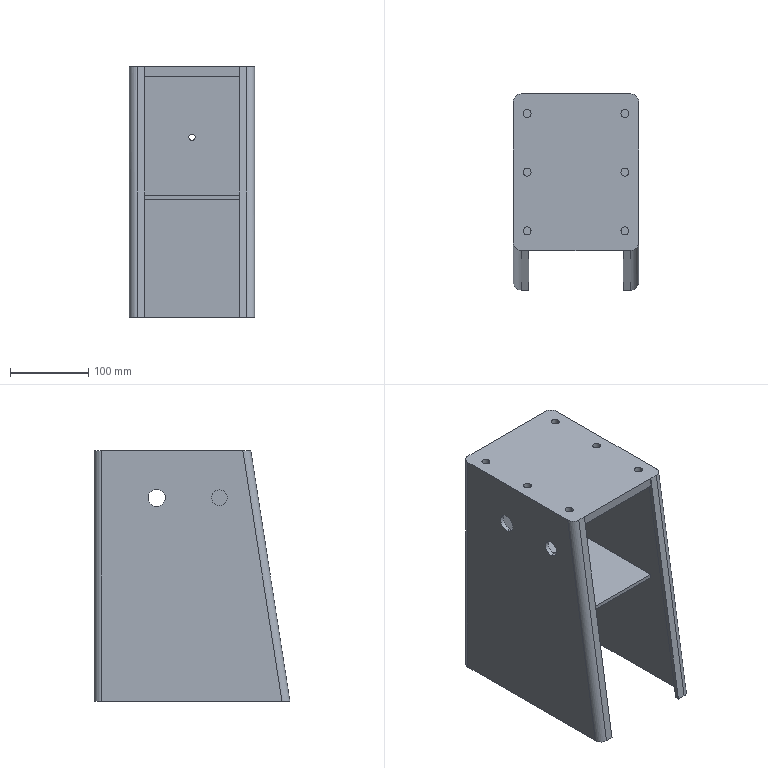Component | SolidWorks | 010MachineHeadWeldedPart-1 | 1 solid | 52 faces | volume 1446415 mm3 | cylinder 32 | plane 20 | commonest cylinder face diameters 10.2 x12 20 x6 10 x6 22 x4 60 x2 8 x2 | material Plain Carbon Steel